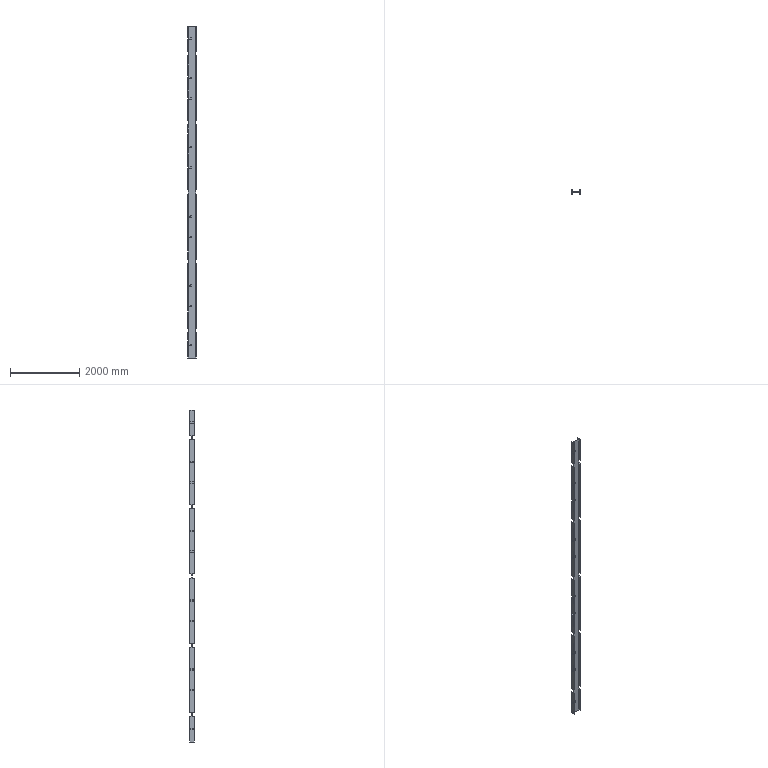Component | NX | CHUNSHUIJINCAO_DI | 1 solid | 214 faces | volume 48554692 mm3 | plane 214